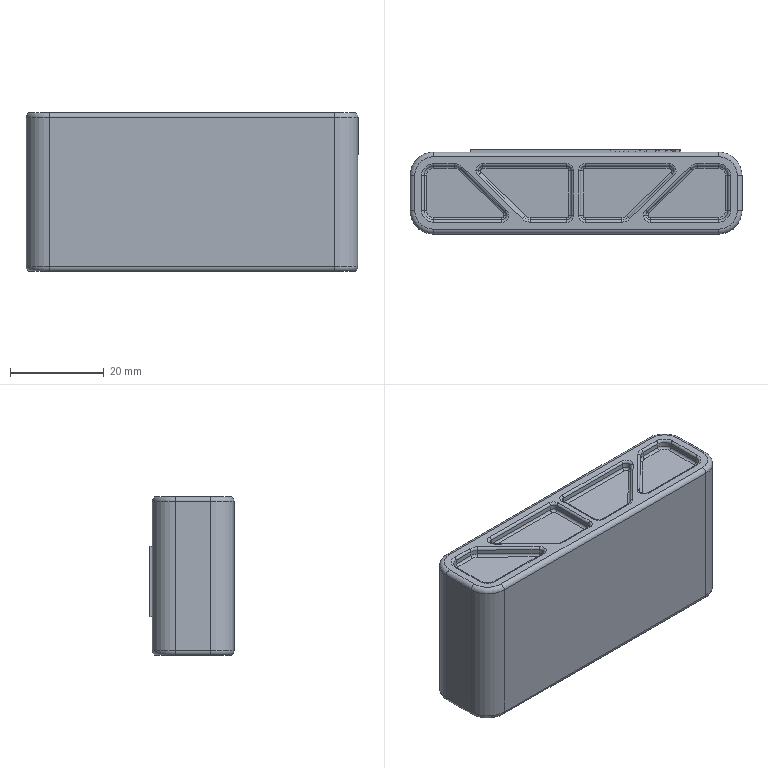Component | SolidWorks | 4.Battery-1 | 1 solid | 410 faces | box 71 x 18 x 34 mm | volume 38985 mm3 | plane 188 | cylinder 112 | torus 84 | spline 26 | commonest cylinder face diameters 1 x64 2 x28 4 x16 10 x4
build123d program:
from build123d import *

# Parameters (mm, degrees)
SKETCH1_W            = 71
SKETCH1_H            = 34
BOSS_EXTRUDE1_DEPTH  = 17.5
FILLET1_R            = 5
FILLET2_R            = 1
SKETCH12_W           = 0.2908
SKETCH12_H           = 1.809
BOSS_EXTRUDE2_DEPTH  = 0.5
CUT_EXTRUDE1_DEPTH   = 2
FILLET3_R            = 0.5
FILLET3_OF_MIRROR1_R = 0.5


with BuildPart() as part:
    # Sketch1 → Boss-Extrude1 (new body)
    with BuildSketch(Plane(origin=(0, 0, 0), x_dir=(1, 0, 0), z_dir=(0, 1, 0))):
        Rectangle(SKETCH1_W, SKETCH1_H)
    extrude(amount=BOSS_EXTRUDE1_DEPTH)

    # Fillet1
    fillet1_edges = [part.edges().sort_by_distance(p)[0] for p in [
        (35.5, 17.5, 0),
        (-35.5, 17.5, 0),
        (35.5, 0, 0),
        (-35.5, 0, 0),
    ]]
    fillet(fillet1_edges, radius=FILLET1_R)

    # Fillet2
    fillet2_edges = [part.edges().sort_by_distance(p)[0] for p in [
        (-35.5, 8.75, 17),
        (-35.5, 8.75, -17),
        (0, 0, 17),
        (35.5, 8.75, 17),
        (0, 17.5, 17),
        (34.036, 16.036, 17),
        (34.036, 1.464, 17),
        (-34.036, 16.036, 17),
        (-34.036, 1.464, 17),
        (0, 0, -17),
        (0, 17.5, -17),
        (35.5, 8.75, -17),
        (34.036, 16.036, -17),
        (34.036, 1.464, -17),
        (-34.036, 16.036, -17),
        (-34.036, 1.464, -17),
    ]]
    fillet(fillet2_edges, radius=FILLET2_R)

    # Sketch12 → Boss-Extrude2 (add)
    # profile 1 of 12: a face of its own
    with BuildSketch(Plane(origin=(0, 17.5, 0), x_dir=(1, 0, 0), z_dir=(0, 1, 0))):
        Polygon((-7.549, 8.661), (-7.549, -1.089), (-5.299, -1.089), (-5.299, 6.411), (20.201, 6.411), (20.201, 1.161), (11.201, 1.161), (11.201, -1.089), (22.451, -1.089), (22.451, 8.661), align=None)
    # profile 2 of 12: a face of its own
    with BuildSketch(Plane(origin=(0, 17.5, 0), x_dir=(1, 0, 0), z_dir=(0, 1, 0))):
        Polygon((-22.549, 8.661), (-22.549, -6.339), (7.451, -6.339), (7.451, 1.161), (-0.04927, 1.161), (-0.04927, -1.089), (5.201, -1.089), (5.201, -4.089), (-20.299, -4.089), (-20.299, 6.411), (-11.299, 6.411), (-11.299, 8.661), align=None)
    # profile 3 of 12: a face of its own
    with BuildSketch(Plane(origin=(0, 17.5, 0), x_dir=(1, 0, 0), z_dir=(0, 1, 0))):
        Polygon((17.312, -6.339), (17.606, -6.339), (17.836, -5.919), (19.048, -5.919), (19.276, -6.339), (19.605, -6.339), (18.61, -4.53), (18.29, -4.53), align=None)
        Polygon((17.961, -5.66), (18.925, -5.66), (18.442, -4.736), align=None, mode=Mode.SUBTRACT)
    # profile 4 of 12: a face of its own
    with BuildSketch(Plane(origin=(0, 17.5, 0), x_dir=(1, 0, 0), z_dir=(0, 1, 0))):
        with BuildLine():
            Line((20.555, -5.076), (21.283, -6.055))
            Line((21.283, -6.055), (21.362, -6.055))
            Line((21.362, -6.055), (22.062, -5.048))
            add(Edge.make_bspline(
                [(22.062, -5.048), (22.07, -5.037), (22.087, -5.012), (22.111, -4.968), (22.14, -4.915), (22.16, -4.875), (22.17, -4.853)],
                knots=[0, 0, 0, 0, 0.1815, 0.4036, 0.676, 1, 1, 1, 1], degree=3))
            add(Edge.make_bspline(
                [(22.17, -4.853), (22.17, -4.862), (22.169, -4.882), (22.168, -4.915), (22.166, -4.955), (22.163, -4.997), (22.161, -5.039), (22.159, -5.073), (22.158, -5.099), (22.158, -5.113), (22.158, -5.118)],
                knots=[0, 0, 0, 0, 0.1028, 0.2266, 0.3752, 0.5467, 0.7106, 0.842, 0.9372, 1, 1, 1, 1], degree=3))
            Line((22.158, -5.118), (22.158, -6.339))
            Line((22.158, -6.339), (22.416, -6.339))
            Line((22.416, -6.339), (22.416, -4.53))
            Line((22.416, -4.53), (22.158, -4.53))
            Line((22.158, -4.53), (21.327, -5.707))
            Line((21.327, -5.707), (20.436, -4.53))
            Line((20.436, -4.53), (20.187, -4.53))
            Line((20.187, -4.53), (20.187, -6.339))
            Line((20.187, -6.339), (20.445, -6.339))
            Line((20.445, -6.339), (20.445, -5.118))
            add(Edge.make_bspline(
                [(20.445, -5.118), (20.446, -5.103), (20.446, -5.074), (20.444, -5.033), (20.444, -4.997), (20.441, -4.956), (20.438, -4.908), (20.434, -4.871), (20.432, -4.853)],
                knots=[0, 0, 0, 0, 0.1711, 0.3251, 0.462, 0.58, 0.7953, 1, 1, 1, 1], degree=3))
            add(Edge.make_bspline(
                [(20.432, -4.853), (20.438, -4.871), (20.451, -4.906), (20.478, -4.959), (20.509, -5.011), (20.534, -5.046), (20.546, -5.064)],
                knots=[0, 0, 0, 0, 0.2318, 0.473, 0.7299, 1, 1, 1, 1], degree=3))
            add(Edge.make_bspline(
                [(20.546, -5.064), (20.548, -5.066), (20.551, -5.07), (20.554, -5.074), (20.555, -5.076)],
                knots=[0, 0, 0, 0, 0.6601, 1, 1, 1, 1], degree=3))
        make_face()
    # profile 5 of 12: a face of its own
    with BuildSketch(Plane(origin=(0, 17.5, 0), x_dir=(1, 0, 0), z_dir=(0, 1, 0))):
        with BuildLine():
            Line((20.445, -3.714), (20.704, -3.714))
            Line((20.704, -3.714), (20.704, -2.648))
            add(Edge.make_bspline(
                [(20.704, -2.648), (20.704, -2.627), (20.703, -2.588), (20.703, -2.531), (20.701, -2.478), (20.698, -2.414), (20.694, -2.339), (20.688, -2.28), (20.685, -2.252)],
                knots=[0, 0, 0, 0, 0.1541, 0.2992, 0.4318, 0.5554, 0.785, 1, 1, 1, 1], degree=3))
            add(Edge.make_bspline(
                [(20.685, -2.252), (20.694, -2.266), (20.714, -2.296), (20.75, -2.339), (20.791, -2.385), (20.823, -2.413), (20.84, -2.429)],
                knots=[0, 0, 0, 0, 0.2173, 0.4547, 0.7153, 1, 1, 1, 1], degree=3))
            add(Edge.make_bspline(
                [(20.84, -2.429), (20.846, -2.434), (20.856, -2.443), (20.867, -2.452), (20.871, -2.456)],
                knots=[0, 0, 0, 0, 0.5858, 1, 1, 1, 1], degree=3))
            Line((20.871, -2.456), (22.277, -3.714))
            Line((22.277, -3.714), (22.448, -3.714))
            Line((22.448, -3.714), (22.448, -1.905))
            Line((22.448, -1.905), (22.19, -1.905))
            Line((22.19, -1.905), (22.19, -2.898))
            add(Edge.make_bspline(
                [(22.19, -2.898), (22.19, -2.924), (22.19, -2.974), (22.191, -3.044), (22.193, -3.105), (22.197, -3.174), (22.204, -3.252), (22.212, -3.312), (22.216, -3.342)],
                knots=[0, 0, 0, 0, 0.1777, 0.3351, 0.4722, 0.589, 0.7981, 1, 1, 1, 1], degree=3))
            add(Edge.make_bspline(
                [(22.216, -3.342), (22.198, -3.32), (22.162, -3.276), (22.108, -3.216), (22.058, -3.161), (22.023, -3.13), (22.007, -3.115)],
                knots=[0, 0, 0, 0, 0.2806, 0.5441, 0.7853, 1, 1, 1, 1], degree=3))
            Line((22.007, -3.115), (20.638, -1.905))
            Line((20.638, -1.905), (20.445, -1.905))
            Line((20.445, -1.905), (20.445, -3.714))
        make_face()
    # profile 6 of 12: a face of its own
    with BuildSketch(Plane(origin=(0, 17.5, 0), x_dir=(1, 0, 0), z_dir=(0, 1, 0))):
        Polygon((13.855, -4.788), (14.695, -4.788), (14.695, -4.53), (12.756, -4.53), (12.756, -4.788), (13.564, -4.788), (13.564, -6.339), (13.855, -6.339), align=None)
    # profile 7 of 12: a face of its own
    with BuildSketch(Plane(origin=(0, 17.5, 0), x_dir=(1, 0, 0), z_dir=(0, 1, 0))):
        Polygon((15.179, -6.339), (16.924, -6.339), (16.924, -6.08), (15.47, -6.08), (15.47, -5.499), (16.342, -5.499), (16.342, -5.24), (15.47, -5.24), (15.47, -4.788), (16.924, -4.788), (16.924, -4.53), (15.179, -4.53), align=None)
    # profile 8 of 12: a face of its own
    with BuildSketch(Plane(origin=(0, 17.5, 0), x_dir=(1, 0, 0), z_dir=(0, 1, 0))):
        with BuildLine():
            Line((19.315, -2.163), (19.315, -2.421))
            Line((19.315, -2.421), (19.605, -2.363))
            Line((19.605, -2.363), (19.605, -2.32))
            add(Edge.make_bspline(
                [(19.605, -2.32), (19.605, -2.301), (19.604, -2.264), (19.601, -2.212), (19.594, -2.165), (19.584, -2.122), (19.572, -2.083), (19.557, -2.049), (19.538, -2.019), (19.517, -1.994), (19.492, -1.972), (19.463, -1.954), (19.428, -1.939), (19.389, -1.925), (19.346, -1.917), (19.298, -1.909), (19.245, -1.906), (19.208, -1.905), (19.189, -1.905)],
                knots=[0, 0, 0, 0, 0.08171, 0.1571, 0.2264, 0.2899, 0.3483, 0.4018, 0.4516, 0.4982, 0.5452, 0.5944, 0.6486, 0.7072, 0.7714, 0.8408, 0.9176, 1, 1, 1, 1], degree=3))
            Line((19.189, -1.905), (18.015, -1.905))
            add(Edge.make_bspline(
                [(18.015, -1.905), (17.996, -1.905), (17.959, -1.906), (17.906, -1.909), (17.857, -1.917), (17.814, -1.927), (17.775, -1.939), (17.741, -1.955), (17.712, -1.974), (17.688, -1.996), (17.667, -2.022), (17.65, -2.054), (17.634, -2.089), (17.623, -2.13), (17.614, -2.175), (17.607, -2.226), (17.603, -2.281), (17.603, -2.32), (17.602, -2.34)],
                knots=[0, 0, 0, 0, 0.08187, 0.1568, 0.2253, 0.2881, 0.345, 0.3979, 0.4462, 0.4916, 0.5371, 0.5868, 0.641, 0.7003, 0.7657, 0.8368, 0.9153, 1, 1, 1, 1], degree=3))
            Line((17.602, -2.34), (17.602, -3.294))
            add(Edge.make_bspline(
                [(17.602, -3.294), (17.603, -3.314), (17.603, -3.351), (17.607, -3.404), (17.613, -3.453), (17.623, -3.497), (17.634, -3.536), (17.65, -3.57), (17.667, -3.6), (17.687, -3.625), (17.712, -3.647), (17.741, -3.665), (17.775, -3.68), (17.814, -3.693), (17.858, -3.702), (17.906, -3.709), (17.959, -3.713), (17.996, -3.713), (18.015, -3.714)],
                knots=[0, 0, 0, 0, 0.08342, 0.1605, 0.2307, 0.2946, 0.3529, 0.4068, 0.4555, 0.5014, 0.5466, 0.5955, 0.6487, 0.7067, 0.7706, 0.8402, 0.9166, 1, 1, 1, 1], degree=3))
            Line((18.015, -3.714), (19.189, -3.714))
            add(Edge.make_bspline(
                [(19.189, -3.714), (19.209, -3.713), (19.246, -3.713), (19.299, -3.709), (19.348, -3.703), (19.391, -3.692), (19.43, -3.681), (19.464, -3.665), (19.494, -3.648), (19.519, -3.626), (19.54, -3.601), (19.558, -3.571), (19.572, -3.537), (19.585, -3.498), (19.594, -3.454), (19.6, -3.405), (19.605, -3.351), (19.605, -3.314), (19.605, -3.294)],
                knots=[0, 0, 0, 0, 0.0831, 0.1592, 0.2292, 0.2929, 0.3505, 0.4035, 0.4525, 0.4981, 0.5442, 0.5932, 0.6459, 0.7051, 0.7694, 0.8394, 0.9162, 1, 1, 1, 1], degree=3))
            Line((19.605, -3.294), (19.605, -2.712))
            Line((19.605, -2.712), (18.572, -2.712))
            Line((18.572, -2.712), (18.572, -2.971))
            Line((18.572, -2.971), (19.315, -2.971))
            Line((19.315, -2.971), (19.315, -3.455))
            Line((19.315, -3.455), (17.893, -3.455))
            Line((17.893, -3.455), (17.893, -2.163))
            Line((17.893, -2.163), (19.315, -2.163))
        make_face()
    # profile 9 of 12: a face of its own
    with BuildSketch(Plane(origin=(0, 17.5, 0), x_dir=(1, 0, 0), z_dir=(0, 1, 0))):
        with Locations((16.52, -2.809)):
            Rectangle(SKETCH12_W, SKETCH12_H)
    # profile 10 of 12: a face of its own
    with BuildSketch(Plane(origin=(0, 17.5, 0), x_dir=(1, 0, 0), z_dir=(0, 1, 0))):
        with BuildLine():
            Line((15.212, -2.163), (15.212, -2.421))
            Line((15.212, -2.421), (15.47, -2.349))
            Line((15.47, -2.349), (15.47, -2.311))
            add(Edge.make_bspline(
                [(15.47, -2.311), (15.47, -2.293), (15.469, -2.258), (15.466, -2.208), (15.457, -2.162), (15.449, -2.12), (15.435, -2.082), (15.42, -2.049), (15.401, -2.02), (15.379, -1.994), (15.353, -1.972), (15.322, -1.955), (15.288, -1.939), (15.248, -1.926), (15.203, -1.916), (15.154, -1.909), (15.101, -1.905), (15.063, -1.905), (15.044, -1.905)],
                knots=[0, 0, 0, 0, 0.07882, 0.1513, 0.2186, 0.2807, 0.3379, 0.3911, 0.4407, 0.4882, 0.5359, 0.5869, 0.6414, 0.7012, 0.767, 0.8385, 0.9161, 1, 1, 1, 1], degree=3))
            Line((15.044, -1.905), (14.071, -1.905))
            add(Edge.make_bspline(
                [(14.071, -1.905), (14.052, -1.905), (14.015, -1.906), (13.962, -1.909), (13.914, -1.917), (13.871, -1.926), (13.832, -1.939), (13.799, -1.955), (13.769, -1.974), (13.745, -1.996), (13.725, -2.022), (13.708, -2.053), (13.693, -2.089), (13.681, -2.13), (13.672, -2.176), (13.666, -2.227), (13.662, -2.283), (13.661, -2.322), (13.661, -2.342)],
                knots=[0, 0, 0, 0, 0.08106, 0.1559, 0.2243, 0.2862, 0.3433, 0.3951, 0.4434, 0.4887, 0.5343, 0.5834, 0.6379, 0.6972, 0.7632, 0.8356, 0.914, 1, 1, 1, 1], degree=3))
            Line((13.661, -2.342), (13.661, -2.493))
            add(Edge.make_bspline(
                [(13.661, -2.493), (13.661, -2.512), (13.662, -2.549), (13.666, -2.602), (13.672, -2.65), (13.681, -2.693), (13.693, -2.732), (13.708, -2.766), (13.725, -2.795), (13.745, -2.82), (13.77, -2.841), (13.799, -2.858), (13.832, -2.874), (13.871, -2.885), (13.914, -2.895), (13.962, -2.901), (14.015, -2.905), (14.052, -2.906), (14.071, -2.906)],
                knots=[0, 0, 0, 0, 0.08353, 0.1599, 0.2302, 0.2938, 0.3529, 0.4057, 0.4543, 0.4996, 0.5448, 0.5938, 0.6469, 0.7053, 0.7691, 0.8393, 0.9165, 1, 1, 1, 1], degree=3))
            Line((14.071, -2.906), (15.244, -2.906))
            Line((15.244, -2.906), (15.244, -3.455))
            Line((15.244, -3.455), (13.855, -3.455))
            Line((13.855, -3.455), (13.855, -3.165))
            Line((13.855, -3.165), (13.596, -3.23))
            Line((13.596, -3.23), (13.596, -3.279))
            add(Edge.make_bspline(
                [(13.596, -3.279), (13.597, -3.299), (13.597, -3.338), (13.601, -3.394), (13.608, -3.444), (13.617, -3.49), (13.628, -3.53), (13.643, -3.566), (13.66, -3.597), (13.681, -3.623), (13.706, -3.645), (13.734, -3.663), (13.768, -3.679), (13.806, -3.692), (13.849, -3.702), (13.896, -3.709), (13.949, -3.713), (13.985, -3.713), (14.004, -3.714)],
                knots=[0, 0, 0, 0, 0.08597, 0.165, 0.2372, 0.3022, 0.3627, 0.417, 0.4664, 0.5122, 0.5574, 0.6061, 0.6583, 0.7151, 0.777, 0.845, 0.919, 1, 1, 1, 1], degree=3))
            Line((14.004, -3.714), (15.07, -3.714))
            add(Edge.make_bspline(
                [(15.07, -3.714), (15.09, -3.713), (15.129, -3.713), (15.184, -3.709), (15.235, -3.702), (15.28, -3.692), (15.321, -3.68), (15.356, -3.664), (15.387, -3.646), (15.413, -3.624), (15.434, -3.598), (15.453, -3.567), (15.468, -3.532), (15.481, -3.491), (15.491, -3.445), (15.498, -3.394), (15.502, -3.338), (15.502, -3.3), (15.502, -3.279)],
                knots=[0, 0, 0, 0, 0.08345, 0.1601, 0.2303, 0.2944, 0.352, 0.4052, 0.4533, 0.4987, 0.5441, 0.5927, 0.6459, 0.7042, 0.7683, 0.8392, 0.9159, 1, 1, 1, 1], degree=3))
            Line((15.502, -3.279), (15.502, -3.074))
            add(Edge.make_bspline(
                [(15.502, -3.074), (15.502, -3.054), (15.501, -3.016), (15.498, -2.961), (15.49, -2.912), (15.481, -2.867), (15.468, -2.827), (15.452, -2.792), (15.433, -2.762), (15.411, -2.736), (15.385, -2.715), (15.354, -2.697), (15.319, -2.681), (15.278, -2.669), (15.233, -2.659), (15.183, -2.652), (15.128, -2.649), (15.09, -2.648), (15.07, -2.648)],
                knots=[0, 0, 0, 0, 0.08303, 0.1592, 0.229, 0.2923, 0.3508, 0.4034, 0.4524, 0.4982, 0.5437, 0.5929, 0.6468, 0.7057, 0.7697, 0.8401, 0.917, 1, 1, 1, 1], degree=3))
            Line((15.07, -2.648), (13.919, -2.648))
            Line((13.919, -2.648), (13.919, -2.163))
            Line((13.919, -2.163), (15.212, -2.163))
        make_face()
    # profile 11 of 12: a face of its own
    with BuildSketch(Plane(origin=(0, 17.5, 0), x_dir=(1, 0, 0), z_dir=(0, 1, 0))):
        Polygon((11.206, -3.714), (12.95, -3.714), (12.95, -3.455), (11.496, -3.455), (11.496, -2.874), (12.369, -2.874), (12.369, -2.615), (11.496, -2.615), (11.496, -2.163), (12.95, -2.163), (12.95, -1.905), (11.206, -1.905), align=None)
    # profile 12 of 12: a face of its own
    with BuildSketch(Plane(origin=(0, 17.5, 0), x_dir=(1, 0, 0), z_dir=(0, 1, 0))):
        with BuildLine():
            Line((9.379, -1.905), (8.395, -1.905))
            Line((8.395, -1.905), (8.395, -3.714))
            Line((8.395, -3.714), (9.379, -3.714))
            add(Edge.make_bspline(
                [(9.379, -3.714), (9.42, -3.713), (9.498, -3.713), (9.609, -3.706), (9.71, -3.696), (9.8, -3.681), (9.882, -3.661), (9.956, -3.637), (10.023, -3.609), (10.063, -3.585), (10.083, -3.573)],
                knots=[0, 0, 0, 0, 0.1681, 0.3213, 0.4603, 0.585, 0.6994, 0.8062, 0.9061, 1, 1, 1, 1], degree=3))
            add(Edge.make_bspline(
                [(10.083, -3.573), (10.112, -3.553), (10.17, -3.513), (10.245, -3.436), (10.311, -3.351), (10.365, -3.254), (10.409, -3.15), (10.44, -3.038), (10.459, -2.92), (10.461, -2.839), (10.463, -2.798)],
                knots=[0, 0, 0, 0, 0.1182, 0.2355, 0.3543, 0.4768, 0.6026, 0.7308, 0.8625, 1, 1, 1, 1], degree=3))
            add(Edge.make_bspline(
                [(10.463, -2.798), (10.461, -2.759), (10.459, -2.682), (10.44, -2.569), (10.408, -2.462), (10.363, -2.359), (10.308, -2.265), (10.243, -2.18), (10.169, -2.105), (10.111, -2.065), (10.083, -2.045)],
                knots=[0, 0, 0, 0, 0.1329, 0.2622, 0.3893, 0.5164, 0.6415, 0.7624, 0.881, 1, 1, 1, 1], degree=3))
            add(Edge.make_bspline(
                [(10.083, -2.045), (10.063, -2.033), (10.022, -2.009), (9.953, -1.98), (9.879, -1.956), (9.797, -1.936), (9.707, -1.922), (9.607, -1.911), (9.497, -1.906), (9.42, -1.905), (9.379, -1.905)],
                knots=[0, 0, 0, 0, 0.0964, 0.1978, 0.3052, 0.4194, 0.5433, 0.6809, 0.8333, 1, 1, 1, 1], degree=3))
        make_face()
        with BuildLine():
            Line((8.686, -2.163), (8.686, -3.455))
            Line((8.686, -3.455), (9.336, -3.455))
            add(Edge.make_bspline(
                [(9.336, -3.455), (9.372, -3.455), (9.44, -3.454), (9.538, -3.447), (9.628, -3.436), (9.71, -3.419), (9.784, -3.397), (9.85, -3.372), (9.908, -3.341), (9.958, -3.305), (10.001, -3.263), (10.039, -3.216), (10.07, -3.161), (10.096, -3.101), (10.115, -3.034), (10.13, -2.962), (10.138, -2.883), (10.139, -2.829), (10.139, -2.801)],
                knots=[0, 0, 0, 0, 0.0881, 0.1697, 0.245, 0.3143, 0.3781, 0.4363, 0.4905, 0.5413, 0.5902, 0.6404, 0.6917, 0.746, 0.8029, 0.8641, 0.9295, 1, 1, 1, 1], degree=3))
            add(Edge.make_bspline(
                [(10.139, -2.801), (10.139, -2.773), (10.138, -2.721), (10.129, -2.644), (10.115, -2.574), (10.095, -2.51), (10.069, -2.451), (10.037, -2.398), (9.999, -2.352), (9.955, -2.311), (9.903, -2.276), (9.845, -2.245), (9.779, -2.22), (9.706, -2.199), (9.624, -2.183), (9.535, -2.171), (9.438, -2.165), (9.371, -2.164), (9.336, -2.163)],
                knots=[0, 0, 0, 0, 0.06894, 0.1331, 0.1935, 0.2497, 0.3032, 0.355, 0.4051, 0.4551, 0.5064, 0.5617, 0.621, 0.6852, 0.755, 0.8305, 0.9119, 1, 1, 1, 1], degree=3))
            Line((9.336, -2.163), (8.686, -2.163))
        make_face(mode=Mode.SUBTRACT)
    extrude(amount=BOSS_EXTRUDE2_DEPTH)

    # Sketch13 → Cut-Extrude1 (cut)
    with BuildSketch(Plane.XY.offset(17)):
        with BuildLine():
            Line((-1, 4), (-1, 13.5))
            ThreePointArc((-1, 13.5), (-1.293, 14.207), (-2, 14.5))
            Line((-2, 14.5), (-19.892, 14.5))
            ThreePointArc((-19.892, 14.5), (-20.818, 13.878), (-20.592, 12.785))
            Line((-20.592, 12.785), (-11.17, 3.57))
            ThreePointArc((-11.17, 3.57), (-10.527, 3.148), (-9.772, 3))
            Line((-9.772, 3), (-2, 3))
            ThreePointArc((-2, 3), (-1.293, 3.293), (-1, 4))
        make_face()
        with BuildLine():
            Line((9.772, 3), (2, 3))
            ThreePointArc((2, 3), (1.293, 3.293), (1, 4))
            Line((1, 4), (1, 13.5))
            ThreePointArc((1, 13.5), (1.293, 14.207), (2, 14.5))
            Line((2, 14.5), (19.892, 14.5))
            ThreePointArc((19.892, 14.5), (20.818, 13.878), (20.592, 12.785))
            Line((20.592, 12.785), (11.17, 3.57))
            ThreePointArc((11.17, 3.57), (10.527, 3.148), (9.772, 3))
        make_face()
        with BuildLine():
            Line((26.021, 14.5), (30.5, 14.5))
            ThreePointArc((30.5, 14.5), (31.914, 13.914), (32.5, 12.5))
            Line((32.5, 12.5), (32.5, 5))
            ThreePointArc((32.5, 5), (31.914, 3.586), (30.5, 3))
            Line((30.5, 3), (15.9, 3))
            ThreePointArc((15.9, 3), (14.974, 3.622), (15.201, 4.715))
            Line((15.201, 4.715), (24.622, 13.93))
            ThreePointArc((24.622, 13.93), (25.266, 14.352), (26.021, 14.5))
        make_face()
        with BuildLine():
            Line((-32.5, 12.5), (-32.5, 5))
            ThreePointArc((-32.5, 5), (-31.914, 3.586), (-30.5, 3))
            Line((-30.5, 3), (-15.9, 3))
            ThreePointArc((-15.9, 3), (-14.974, 3.622), (-15.201, 4.715))
            Line((-15.201, 4.715), (-24.622, 13.93))
            ThreePointArc((-24.622, 13.93), (-25.266, 14.352), (-26.021, 14.5))
            Line((-26.021, 14.5), (-30.5, 14.5))
            ThreePointArc((-30.5, 14.5), (-31.914, 13.914), (-32.5, 12.5))
        make_face()
    cut_extrude1 = extrude(amount=-CUT_EXTRUDE1_DEPTH, mode=Mode.SUBTRACT)

    # Fillet3
    fillet3_edges = [part.edges().sort_by_distance(p)[0] for p in [
        (-20.818, 13.878, 15),
        (-10.946, 14.5, 15),
        (-1.293, 14.207, 15),
        (-1, 8.75, 15),
        (-1.293, 3.293, 15),
        (-5.886, 3, 15),
        (-10.527, 3.148, 15),
        (-15.881, 8.178, 15),
        (-20.818, 13.878, 17),
        (-15.881, 8.178, 17),
        (-10.527, 3.148, 17),
        (-5.886, 3, 17),
        (-1.293, 3.293, 17),
        (-1, 8.75, 17),
        (-1.293, 14.207, 17),
        (-10.946, 14.5, 17),
        (-31.914, 13.914, 15),
        (-28.26, 14.5, 15),
        (-25.266, 14.352, 15),
        (-19.912, 9.322, 15),
        (-14.974, 3.622, 15),
        (-23.2, 3, 15),
        (-31.914, 3.586, 15),
        (-32.5, 8.75, 15),
        (-31.914, 13.914, 17),
        (-32.5, 8.75, 17),
        (-31.914, 3.586, 17),
        (-23.2, 3, 17),
        (-14.974, 3.622, 17),
        (-19.912, 9.322, 17),
        (-25.266, 14.352, 17),
        (-28.26, 14.5, 17),
        (10.527, 3.148, 15),
        (5.886, 3, 15),
        (1.293, 3.293, 15),
        (1, 8.75, 15),
        (1.293, 14.207, 15),
        (10.946, 14.5, 15),
        (20.818, 13.878, 15),
        (15.881, 8.178, 15),
        (10.527, 3.148, 17),
        (15.881, 8.178, 17),
        (20.818, 13.878, 17),
        (10.946, 14.5, 17),
        (1.293, 14.207, 17),
        (1, 8.75, 17),
        (1.293, 3.293, 17),
        (5.886, 3, 17),
        (31.914, 3.586, 15),
        (23.2, 3, 15),
        (14.974, 3.622, 15),
        (19.912, 9.322, 15),
        (25.266, 14.352, 15),
        (28.26, 14.5, 15),
        (31.914, 13.914, 15),
        (32.5, 8.75, 15),
        (31.914, 3.586, 17),
        (32.5, 8.75, 17),
        (31.914, 13.914, 17),
        (28.26, 14.5, 17),
        (25.266, 14.352, 17),
        (19.912, 9.322, 17),
        (14.974, 3.622, 17),
        (23.2, 3, 17),
    ]]
    fillet(fillet3_edges, radius=FILLET3_R)

    # Mirror1: Cut-Extrude1 across plane
    add(cut_extrude1.mirror(Plane.XY), mode=Mode.SUBTRACT)

    # Fillet3 of Mirror1
    fillet3_of_mirror1_edges = [part.edges().sort_by_distance(p)[0] for p in [
        (-20.818, 13.878, -15),
        (-10.946, 14.5, -15),
        (-1.293, 14.207, -15),
        (-1, 8.75, -15),
        (-1.293, 3.293, -15),
        (-5.886, 3, -15),
        (-10.527, 3.148, -15),
        (-15.881, 8.178, -15),
        (-20.818, 13.878, -17),
        (-15.881, 8.178, -17),
        (-10.527, 3.148, -17),
        (-5.886, 3, -17),
        (-1.293, 3.293, -17),
        (-1, 8.75, -17),
        (-1.293, 14.207, -17),
        (-10.946, 14.5, -17),
        (-31.914, 13.914, -15),
        (-28.26, 14.5, -15),
        (-25.266, 14.352, -15),
        (-19.912, 9.322, -15),
        (-14.974, 3.622, -15),
        (-23.2, 3, -15),
        (-31.914, 3.586, -15),
        (-32.5, 8.75, -15),
        (-31.914, 13.914, -17),
        (-32.5, 8.75, -17),
        (-31.914, 3.586, -17),
        (-23.2, 3, -17),
        (-14.974, 3.622, -17),
        (-19.912, 9.322, -17),
        (-25.266, 14.352, -17),
        (-28.26, 14.5, -17),
        (10.527, 3.148, -15),
        (5.886, 3, -15),
        (1.293, 3.293, -15),
        (1, 8.75, -15),
        (1.293, 14.207, -15),
        (10.946, 14.5, -15),
        (20.818, 13.878, -15),
        (15.881, 8.178, -15),
        (10.527, 3.148, -17),
        (15.881, 8.178, -17),
        (20.818, 13.878, -17),
        (10.946, 14.5, -17),
        (1.293, 14.207, -17),
        (1, 8.75, -17),
        (1.293, 3.293, -17),
        (5.886, 3, -17),
        (31.914, 3.586, -15),
        (23.2, 3, -15),
        (14.974, 3.622, -15),
        (19.912, 9.322, -15),
        (25.266, 14.352, -15),
        (28.26, 14.5, -15),
        (31.914, 13.914, -15),
        (32.5, 8.75, -15),
        (31.914, 3.586, -17),
        (32.5, 8.75, -17),
        (31.914, 13.914, -17),
        (28.26, 14.5, -17),
        (25.266, 14.352, -17),
        (19.912, 9.322, -17),
        (14.974, 3.622, -17),
        (23.2, 3, -17),
    ]]
    fillet(fillet3_of_mirror1_edges, radius=FILLET3_OF_MIRROR1_R)


solid = part.part

# Placed as in the assembly
solid = solid.moved(Location((0, 28.1, 0), (0, 0, 0)))